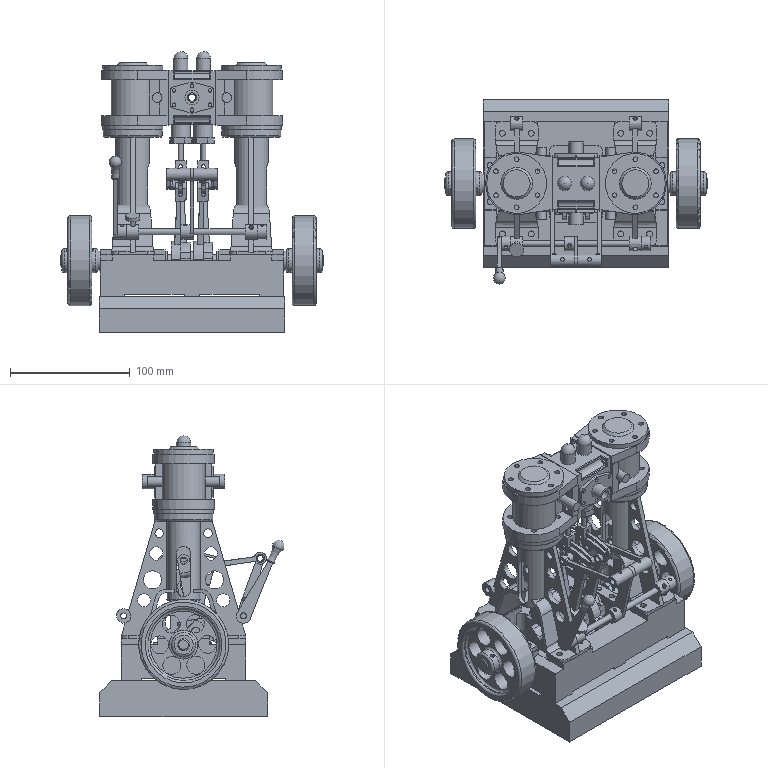Assembly | NX | mm | 127 component files | 134 solids | 2203 faces | box 219 x 154.03 x 234.5 mm | volume 1428194 mm3 | plane 1155 | cylinder 974 | torus 49 | cone 18 | spline 4 | sphere 3 | commonest cylinder face diameters 4 x137 3 x117 8 x68 12 x68 6 x58 5 x57 2.5 x46 10 x45
Bill of materials:
unnamed part 1 | 3 |  | Short cylindrical disc with a recessed band around its outer edge, so it looks like a spool or pulley with two flanges. It has a large off-center through-bore and a small through-hole near the rim.
unnamed part 2 | 4 |  | Half-ring (semicircular saddle) body with flat rectangular tabs at both ends. Each tab has a vertical through-hole. A raised center band runs along the inside of the arc, and the tabs have stepped notches where the band meets them.
unnamed part 3 | 1 |  | Wheel with a wide, rounded-edge rim, a web with six circular lightening holes, and a central hub with a through-bore. The hub sticks out past both faces of the rim. There is a small radial hole in the hub.
unnamed part 4 | 1 |  | Long, slender solid cylindrical rod. It has a transverse cross hole near each end and a short flat or notch at mid-length.
unnamed part 5 | 1 |  | Thick rectangular plate with chamfers along two opposite top edges and six small through-holes arranged in a 2 x 3 grid.
unnamed part 6 | 2 |  | Obround (stadium-shaped) block with two large parallel through-holes through its thickness. The long flat side faces each have two smaller holes that run perpendicular to the large holes and appear to break into them.
unnamed part 7 | 2 |  | Circular flange with four through-holes on a bolt circle and a central through-bore. One face has a short raised boss with a partial-arc edge and a small semicircular notch. The other face has a longer cylindrical spigot joined to the flange by a chamfer.
unnamed part 8 | 4 |  | Solid stepped cylindrical pin: a longer, larger-diameter body with a shorter, smaller-diameter coaxial stub at one end.
unnamed part 9 | 1 |  | Flat tapered lever arm. The narrow end is a thin ring eye around a larger hole. The wider rounded end has a smaller hole and a cylindrical hub boss that projects to one side. The hub has a radial cross hole.
unnamed part 10 | 1 |  | Solid T-shaped or mushroom-shaped part: a flat circular head disc with a smaller-diameter coaxial cylindrical shank.
unnamed part 11 | 2 |  | Elongated arm with a fork (clevis) at one end, made of two parallel lugs with cross holes. The shank tapers toward the other end, which has a semicircular saddle cutout with small tabs or bosses on either side.
unnamed part 12 | 2 |  | Circular flange with six through-holes on a bolt circle and a solid center. One face has a raised central boss with a chamfered edge. The other face has a short cylindrical spigot.
unnamed part 13 | 4 |  | Tapered arm or strut that ends in a forked (clevis-like) tab at the top and a half-ring (semicircular saddle) base at the bottom, with a flat flange on each side of the arch.
unnamed part 14 | 4 |  | Short thick-walled cylinder (collar or bushing form) with a central axial bore and one radial hole through the side wall.
unnamed part 15 | 1 |  | Rectangular frame-like block with three rounded-rectangle through-openings. Raised pads on the top carry drilled holes, and the top and bottom edges have stepped profiles.
unnamed part 16 | 1 |  | Short thick-walled cylinder with a central axial bore and a cylindrical pin set crosswise through the wall and bore. The pin ends sit slightly proud of the outer surface.
unnamed part 17 | 2 |  | Flat plate shaped as a half-round end joined to a tapered straight end. It has a large central through-hole, a ring of smaller through-holes around it, and side holes drilled into the flat end face.
unnamed part 18 | 2 |  | Hexagonal base with a cylindrical boss rising from it and a central through-bore, similar in form to a flanged hex standoff or spacer.
unnamed part 19 | 2 |  | Plain solid cylindrical rod or pin with flat ends.
unnamed part 20 | 1 |  | Crank-handle form: a tapered flat arm with a rounded hub at one end and a turned, knob-like grip at the other.
unnamed part 21 | 2 |  | Disc-shaped cylinder with a small central through-hole and several shallow circumferential grooves around its outer surface, forming a stack of ribs.
unnamed part 22 | 2 |  | Half-bearing or clamp-cap style block with a semicircular cradle between two flat ears, each ear carrying a through-hole. A small pin or locating stub projects inside the cradle.
unnamed part 23 | 2 |  | Stepped cylindrical sleeve with a large through-bore. It has a wider central band with a flat on one side and narrower ends, each with rectangular slots or notches.
unnamed part 24 | 2 |  | Thin flat square plate with corner holes, a second set of larger holes, and three central slots.
unnamed part 25 | 4 |  | Flat, tapered plate shaped like an arm, with four through-holes of different sizes in a row and a semicircular notch on one edge.
unnamed part 26 | 2 |  | Flat, curved plate with a long arc-shaped slot along its upper band and three lobes with round holes along its lower edge.
unnamed part 27 | 1 |  | Solid cylindrical pin with a stepped-down smaller-diameter end. A short cross pin passes through the reduced end and sticks out on both sides.
unnamed part 28 | 2 |  | Symmetric stepped cylindrical shaft with a larger central collar section and two smaller-diameter ends. Each end carries a short cross pin that sticks out on both sides.
unnamed part 29 | 4 |  | Bent strip bracket with an S/Z-shaped (joggled) profile: a flat base flange with two holes, an inclined web, and an upper flange with a concave arc-shaped cut-out at its free edge.
unnamed part 30 | 2 |  | Flanged tubular sleeve: a round flange with four small holes and a counterbored or chamfered central bore, a hollow cylindrical body below it, and a long slot through the tube wall.
unnamed part 31 | 2 |  | Stepped hollow bushing: a cylinder with a larger and a smaller outside diameter and a constant through-bore.
unnamed part 32 | 1 |  | Long slender stepped shaft with smaller-diameter journals at both ends. Each journal has a short cross pin that sticks out on both sides.
unnamed part 33 | 2 |  | Short cylindrical block with an axial through-bore, one flat machined along its side, and a radial cross-hole through the side.
unnamed part 34 | 2 |  | Cylindrical block with two parallel opposite side slots that leave an I-shaped (spool-like) cross-section. It has an axial hole through the central web and a larger cross-hole through the web.
unnamed part 35 | 2 |  | Flat plate with one rounded end and one squared, tapered end. It has a large central bore with a small edge notch, a ring of eight small through-holes, and small holes drilled into the flat end edge.
unnamed part 36 | 2 |  | Slender cylindrical rod attached to a rectangular clevis-like end block. The block has a slot and a cross-hole and a rounded lower end.
unnamed part 37 | 2 |  | Open semi-cylindrical shell (trough/half-sleeve) with uniform wall thickness, flat rectangular top edges, and a single radial through-hole at the bottom center of the curved wall.
unnamed part 38 | 2 |  | Flat plate of uniform thickness with an elongated hexagonal outline and rounded corners, a large central circular through-hole, and six smaller through-holes around it.
unnamed part 39 | 2 |  | Solid stepped round pin: a larger-diameter cylinder with a hemispherical or domed end, and a smaller-diameter coaxial cylindrical shank at the other end.
unnamed part 40 | 4 |  | Thin curved strip shaped as a semicircular arc with a rectangular cross-section, with flat cut ends and no visible holes.
unnamed part 41 | 4 |  | Thin curved ring segment shaped as a semicircular arc with a rectangular cross-section; its radial wall is thinner relative to its radius than in the similar arc part.
unnamed part 42 | 2 |  | Slender stepped cylindrical shaft/pin with a longer, larger-diameter central section and a shorter, reduced-diameter coaxial journal at each end.
unnamed part 43 | 1 |  | Link/crank-arm shaped part: a straight flat bar joining two hollow cylindrical bosses whose axes are parallel to each other. The larger boss has a plain bore. The smaller boss has a reduced-diameter tubular spigot on one side. Each boss has a small radial cross-hole.
unnamed part 44 | 4 |  | Rectangular flat bar with two through-holes near its ends and a smaller countersunk hole at the center. On the underside, two short legs form a central semicircular saddle cut-out.
unnamed part 45 | 1 |  | Link/crank-arm part like the other link: a flat bar joining a larger hollow cylindrical boss and a smaller hollow boss with a stepped tubular spigot. Both bosses have small radial cross-holes; the spigot is on the opposite (mirrored) side.
unnamed part 46 | 1 |  | Plain straight round tube with constant outer and inner diameters and flat square-cut ends.
unnamed part 47 | 4 |  | Rectangular block with a semicircular cradle cut into its top face along the full length, and one through-hole at the bottom of the cradle running down through the base.
unnamed part 48 | 4 |  | Spool-like flanged sleeve: a cylindrical body with a through-bore, a raised flange at each end, and a small radial hole through the middle of the body wall.
unnamed part 49 | 1 |  | Plain flat ring: short hollow cylinder with a central through bore, flat parallel faces and a fairly thick wall.
unnamed part 50 | 1 |  | Wheel-like disc: wide cylindrical rim with rounded edges, a recessed web with six circular lightening holes in a ring, and a central hub with a bore that sticks out on both sides.
unnamed part 51 | 1 |  | Roughly cubic open frame or block. Opposite faces carry flanges with a pattern of small through holes and large rounded-rectangle windows. One face has two larger round holes, and part-cylindrical channels run along the edges between the flanges.
unnamed part 52 | 1 |  | Stepped cylindrical pin or shaft: a long main body with a chamfered end and a shorter, smaller-diameter end section. A short cross pin passes through the small section and sticks out on both sides.
unnamed part 53 | 2 |  | Prismatic block with a forked, U-shaped profile: a solid rectangular body with two parallel prongs extending from it, and a rectangular pocket or window recessed into one side face.
unnamed part 54 | 2 |  | Stepped cylindrical bushing: a larger-diameter base cylinder with a coaxial smaller-diameter cylinder on top and a single through bore along the axis.
unnamed part 55 | 1 |  | Grooved circular disc, similar to a pulley: a cylinder with a circumferential groove between two flanges, a large through bore that is off-centre, a small axial through hole near the rim, and a small radial hole in the bottom of the groove.
unnamed part 56 | 2 |  | Thin conical or dished washer-like disc: a flat circular base, a conical top surface rising to a flat annular land, and a central through hole.
unnamed part 57 | 2 |  | Thick plain ring or spacer: a short hollow cylinder with a central through bore and flat end faces.
unnamed part 58 | 2 |  | Rectangular plate with a raised rectangular boss or tab on its back face. The plate has four corner through holes, two outer slots, and a central keyhole-like slot. A cross hole passes through the boss parallel to the plate, and there is a semicircular notch on one edge.
unnamed part 59 | 2 |  | Oblong link or bar with rounded ends. Two large through holes run through its thickness, each with a stepped smaller hole inside, and two small holes enter the long side face at right angles to them.
unnamed part 60 | 2 |  | Part-cylindrical shell (curved half-sleeve) of uniform wall thickness, covering an arc a little over 180 degrees, with one radial through hole near the middle of the outer surface.
unnamed part 61 | 2 |  | Hexagonal flange base with a coaxial cylindrical boss rising from one face; a single small round bore runs through the full length along the central axis.
Mates:
1. fix | 01__27 1 component
2. touch align | 02B__27 4 face | 02D__27 4 face
3. center | 02B__27 4 face | 02B__27 4 face | 02D__27 4 face | 02D__27 4 face
4. touch align | 02B__27 4 edge | 02D__27 4 face
5. concentric | 02D__27 4 edge | 01__27 1 edge
6. concentric | 02D__27 4 edge | 01__27 1 edge
7. touch align | 02A__27 2 face | 02D__27 4 face
8. touch align | 02A__27 2 face | 02B__27 4 face
9. touch align | 03A__27 2 face | 03D__27 2 face
10. touch align | 03A__27 2 face | 03D__27 2 face
11. touch align | 03A__27 2 face | 03D__27 2 face
12. parallel | 02A__27 2 face | 01__27 1 face
13. concentric | 03A__27 2 edge | 03C__27 2 arc
14. touch align | 03D__27 2 face | 03C__27 2 face
15. parallel | 03D__27 2 face | 01__27 1 face
16. concentric | 03B__27 2 arc | 03A__27 2 edge
17. touch align | 03C__27 2 face | 03B__27 2 face
18. touch align | 03E__27 2 face | 03D__27 2 face
19. center | 03D__27 2 face | 03D__27 2 face | 03E__27 2 face | 03E__27 2 face
20. touch align | 02C__27 4 face | 02B__27 4 face
21. center | 02B__27 4 face | 02B__27 4 face | 02C__27 4 face | 02C__27 4 face
22. concentric | 05A__27 1 edge | 04__27 1 edge
23. concentric | 05A__27 1 edge | 04__27 1 edge
24. concentric | 05B__27 1 edge | 05A__27 1 edge
25. concentric | 05B__27 2 edge | 05A__27 1 edge
26. concentric | 06__27 2 edge | 03B__27 2 edge
27. touch align | 06__27 2 face | 03A__27 2 face
28. concentric | 07__27 2 edge | 02A__27 2 edge
29. concentric | 07__27 2 edge | 02A__27 2 edge
30. touch align | 03A__27 2 face | 07__27 2 face
31. touch align | 03C__27 2 face | 07__27 2 face
32. concentric | 05E__27 2 edge | 05A__27 1 edge
33. concentric | 04__27 2 edge | 03B__27 2 edge
34. concentric | 04__27 2 edge | 03D__27 2 edge
35. concentric | 05A__27 1 edge | 04__27 2 edge
36. parallel | 05A__27 1 face | 01__27 1 face
37. concentric | 05E__27 2 edge | 05A__27 1 edge
38. concentric | 05D__27 2 edge | 05E__27 2 edge
39. concentric | 05C__27 2 edge | 05A__27 1 edge
40. concentric | 05C__27 1 edge | 05A__27 1 edge
41. concentric | 05D__27 1 edge | 05E__27 1 edge
42. concentric | 10__27 2 edge | 08__27 2 edge
43. concentric | 10__27 2 edge | 07__27 2 edge
44. concentric | 11__27 2 edge | 09__27 2 edge
45. concentric | 11__27 2 edge | 05C__27 1 edge
46. concentric | 09__27 1 edge | 11__27 1 edge
47. concentric | 11__27 1 edge | 05C__27 2 edge
48. concentric | 10__27 1 edge | 08__27 1 edge
49. concentric | 10__27 1 edge | 07__27 1 edge
50. concentric | 12A__27 4 edge | 12B__27 4 edge
51. parallel | 12B__27 4 face | 12A__27 4 face
52. concentric | 13__27 4 edge | 12A__27 4 edge
53. touch align | 12B__27 4 face | 13__27 4 face
54. touch align | 14__27 4 face | 13__27 4 face
55. touch align | 13__27 4 face | 14__27 4 face
56. concentric | 12B__27 4 edge | 01__27 1 edge
57. concentric | 12B__27 4 edge | 01__27 1 edge
58. fix | assembly component
59. bond | 12B__27 4 component | assembly component
60. bond | 13__27 4 component | assembly component
61. bond | 12A__27 4 component | assembly component
62. bond | 14__27 4 component | assembly component
63. bond | 12B__27 3 component | assembly component
64. bond | 13__27 3 component | assembly component
65. bond | 12A__27 3 component | assembly component
66. bond | 14__27 3 component | assembly component
67. touch align | 22B__27 2 face | 22A__27 2 face
68. touch align | 22A__27 2 face | 22B__27 2 face
69. center | 22A__27 2 face | 22A__27 2 face | 22B__27 2 datumplane
70. touch align | 22C__27 2 face | 22B__27 2 face
71. concentric | 18B__27 2 edge | 18C__27 2 edge
72. concentric | 18A__27 2 edge | 18B__27 2 edge
73. concentric | 15D__27 2 edge | 15A__27 4 edge
74. touch align | 15B__27 2 face | 15A__27 4 face
75. touch align | 15B__27 2 face | 15A__27 4 face
76. touch align | 15D__27 2 face | 15A__27 3 face
77. touch align | 15A__27 3 face | 15D__27 2 face
78. touch align | 15C__27 1 face | 15A__27 3 face
79. touch align | 15C__27 1 face | 15A__27 3 face
80. concentric | 17C__27 4 edge | 17A__27 2 edge
81. concentric | 17C__27 3 edge | 17B__27 2 edge
82. touch align | 17A__27 2 face | 17C__27 4 face
83. touch align | 17B__27 2 face | 17C__27 3 face
84. concentric | 17B__27 2 edge | 17A__27 2 edge
85. touch align | 17B__27 2 face | 17A__27 2 face
86. touch align | 17C__27 3 face | 15D__27 2 face
87. center | 17A__27 2 face | 17A__27 2 face | 15A__27 4 face | 15A__27 3 face
88. touch align | 18C__27 2 face | 17A__27 2 face
89. center | 17A__27 2 face | 17A__27 2 face | 18C__27 2 face | 18C__27 2 face
90. touch align | 19__27 2 face | 15B__27 2 face
91. concentric | 19__27 2 edge | 15B__27 2 edge
92. touch align | 15B__27 2 face | 13__27 1 face
93. fix | 12B__27 1 component
94. fix | 13__27 1 component
95. fix | 12A__27 2 component
96. fix | 12A__27 1 component
97. fix | 13__27 2 component
98. fix | 12B__27 2 component
99. fix | 14__27 2 component
100. fix | 14__27 1 component
101. center | 17B__27 2 face | 17B__27 2 face | 01__27 1 face | 01__27 1 face
102. touch align | 18B__27 2 face | 07__27 1 face
103. touch align | 18B__27 2 face | 03A__27 1 face
104. fix | 07__27 1 component
105. fix | 06__27 1 component
106. fix | 03B__27 1 component
107. fix | 03C__27 1 component
108. fix | 02D__27 1 component
109. fix | 02B__27 2 component
110. fix | 02D__27 2 component
111. fix | 02B__27 1 component
112. fix | 02A__27 1 component
113. touch align | 22C__27 2 face | 09__27 1 face
114. parallel | 22A__27 2 face | 02B__27 2 face
115. concentric | 20C__27 8 edge | 20A__27 4 edge
116. concentric | 20B__27 4 edge | 20A__27 4 edge
117. concentric | 20B__27 4 edge | 20A__27 4 edge
118. touch align | 20C__27 8 face | 20C__27 7 face
119. concentric | 20C__27 7 edge | 20B__27 4 edge
120. concentric | 24__27 1 edge | 01__27 1 edge
121. concentric | 24__27 1 edge | 01__27 1 edge
122. touch align | 23E__27 1 face | 23B__27 1 face
123. touch align | 23E__27 1 face | 23B__27 1 face
124. touch align | 23A__27 1 face | 23B__27 1 face
125. touch align | 23B__27 1 face | 23A__27 1 face
126. concentric | 23D__27 2 edge | 23C__27 1 edge
127. concentric | 23D__27 1 edge | 23C__27 1 edge
128. touch align | 23D__27 2 face | 23D__27 1 face
129. touch align | 23C__27 1 face | 23B__27 1 face
130. concentric | 23F__27 1 edge | 23D__27 1 edge
131. concentric | 16B__27 4 edge | 20C__27 7 edge
132. concentric | 23A__27 1 edge | 02C__27 1 edge
133. touch align | 02C__27 1 face | 02B__27 2 face
134. center | 02B__27 2 face | 02B__27 2 face | 02C__27 1 face | 02C__27 1 face
135. touch align | 23G__27 1 face | 02C__27 1 face
136. touch align | 22B__27 1 face | 22A__27 1 face
137. touch align | 22B__27 1 face | 22A__27 1 face
138. center | 22A__27 1 face | 22A__27 1 face | 22B__27 1 face
139. touch align | 22C__27 1 face | 22B__27 1 face
140. concentric | 17A__27 1 edge | 17B__27 1 edge
141. touch align | 17A__27 1 face | 17B__27 1 face
142. concentric | 17C__27 2 edge | 17A__27 1 edge
143. touch align | 17C__27 2 face | 17B__27 1 face
144. concentric | 17C__27 1 edge | 17B__27 1 edge
145. touch align | 17B__27 1 edge | 17C__27 1 face
146. concentric | 18A__27 1 edge | 18B__27 1 edge
147. concentric | 18B__27 1 edge | 18C__27 1 edge
148. touch align | 17A__27 1 face | 18C__27 1 face
149. center | 17A__27 1 face | 17A__27 1 face | 18C__27 1 face | 18C__27 1 face
150. touch align | 18B__27 1 face | 02A__27 2 face
151. concentric | 15A__27 2 edge | 15C__27 1 edge
152. touch align | 15C__27 1 face | 15A__27 2 face
153. touch align | 15A__27 2 face | 17C__27 1 face
154. touch align | 15D__27 1 face | 15A__27 2 face
155. touch align | 15D__27 1 face | 17C__27 1 face
156. touch align | 15A__27 1 face | 15D__27 1 face
157. touch align | 15A__27 1 face | 15D__27 1 face
158. touch align | 15B__27 1 face | 15A__27 1 face
159. touch align | 15B__27 1 face | 15A__27 1 face
160. concentric | 19__27 1 edge | 15B__27 1 edge
161. touch align | 15B__27 1 face | 13__27 4 face
162. concentric | 20B__27 3 edge | 20A__27 2 edge
163. concentric | 20B__27 3 edge | 20A__27 2 edge
164. concentric | 20B__27 2 edge | 20A__27 3 edge
165. concentric | 20A__27 3 edge | 20B__27 2 edge
166. concentric | 20B__27 1 edge | 20A__27 1 edge
167. concentric | 20A__27 1 edge | 20B__27 1 edge
168. concentric | 16B__27 2 edge | 20B__27 3 edge
169. concentric | 16B__27 1 edge | 20B__27 1 edge
170. concentric | 16B__27 3 edge | 20B__27 2 edge
171. concentric | 20C__27 4 edge | 20C__27 2 edge
172. concentric | 20C__27 3 edge | 20C__27 5 edge
173. concentric | 20C__27 1 edge | 20C__27 6 edge
174. concentric | 20C__27 6 edge | 20B__27 2 edge
175. concentric | 20C__27 5 edge | 20B__27 3 edge
176. concentric | 20C__27 2 edge | 20B__27 1 edge
177. concentric | 16B__27 1 edge | 16B__27 4 edge
178. concentric | 16B__27 3 edge | 16B__27 2 edge
179. parallel | 20A__27 1 face | 20A__27 2 face
180. parallel | 20A__27 4 face | 20A__27 3 face
181. touch align | 21__27 2 face | 20A__27 1 face
182. touch align | 21__27 2 face | 20A__27 4 face
183. center | 21__27 2 face | 21__27 2 face | 20A__27 1 face | 20A__27 1 face
184. concentric | 16C__27 1 edge | 16B__27 3 edge
185. concentric | 16B__27 1 edge | 16C__27 1 edge
186. center | 21__27 2 face | 21__27 2 face | 22C__27 2 face | 22C__27 2 face
187. touch align | 22C__27 1 face | 09__27 2 face
188. parallel | 22A__27 1 face | 05A__27 1 face
189. center | 21__27 1 face | 21__27 1 face | 22C__27 1 face | 22C__27 1 face
190. parallel | 22C__27 1 face | 22C__27 2 face
191. touch align | 21__27 1 face | 20A__27 2 face
192. touch align | 20A__27 3 face | 21__27 1 face
193. parallel | 20B__27 3 face | 01__27 1 face
194. touch align | 16B__27 2 face | 15C__27 1 face
195. concentric | 23D__27 1 edge | 21__27 1 edge
196. concentric | 23D__27 2 edge | 21__27 2 edge
197. touch align | 03A__27 1 face | 03D__27 1 face
198. touch align | 03D__27 1 face | 04__27 1 face
199. concentric | 03A__27 1 edge | 03B__27 1 edge
200. touch align | 03D__27 1 face | 03B__27 1 face
201. touch align | 22C__27 2 face | 21__27 2 face
202. touch align | 22C__27 1 face | 21__27 1 face
203. touch align | 03A__27 1 face | 03D__27 1 face